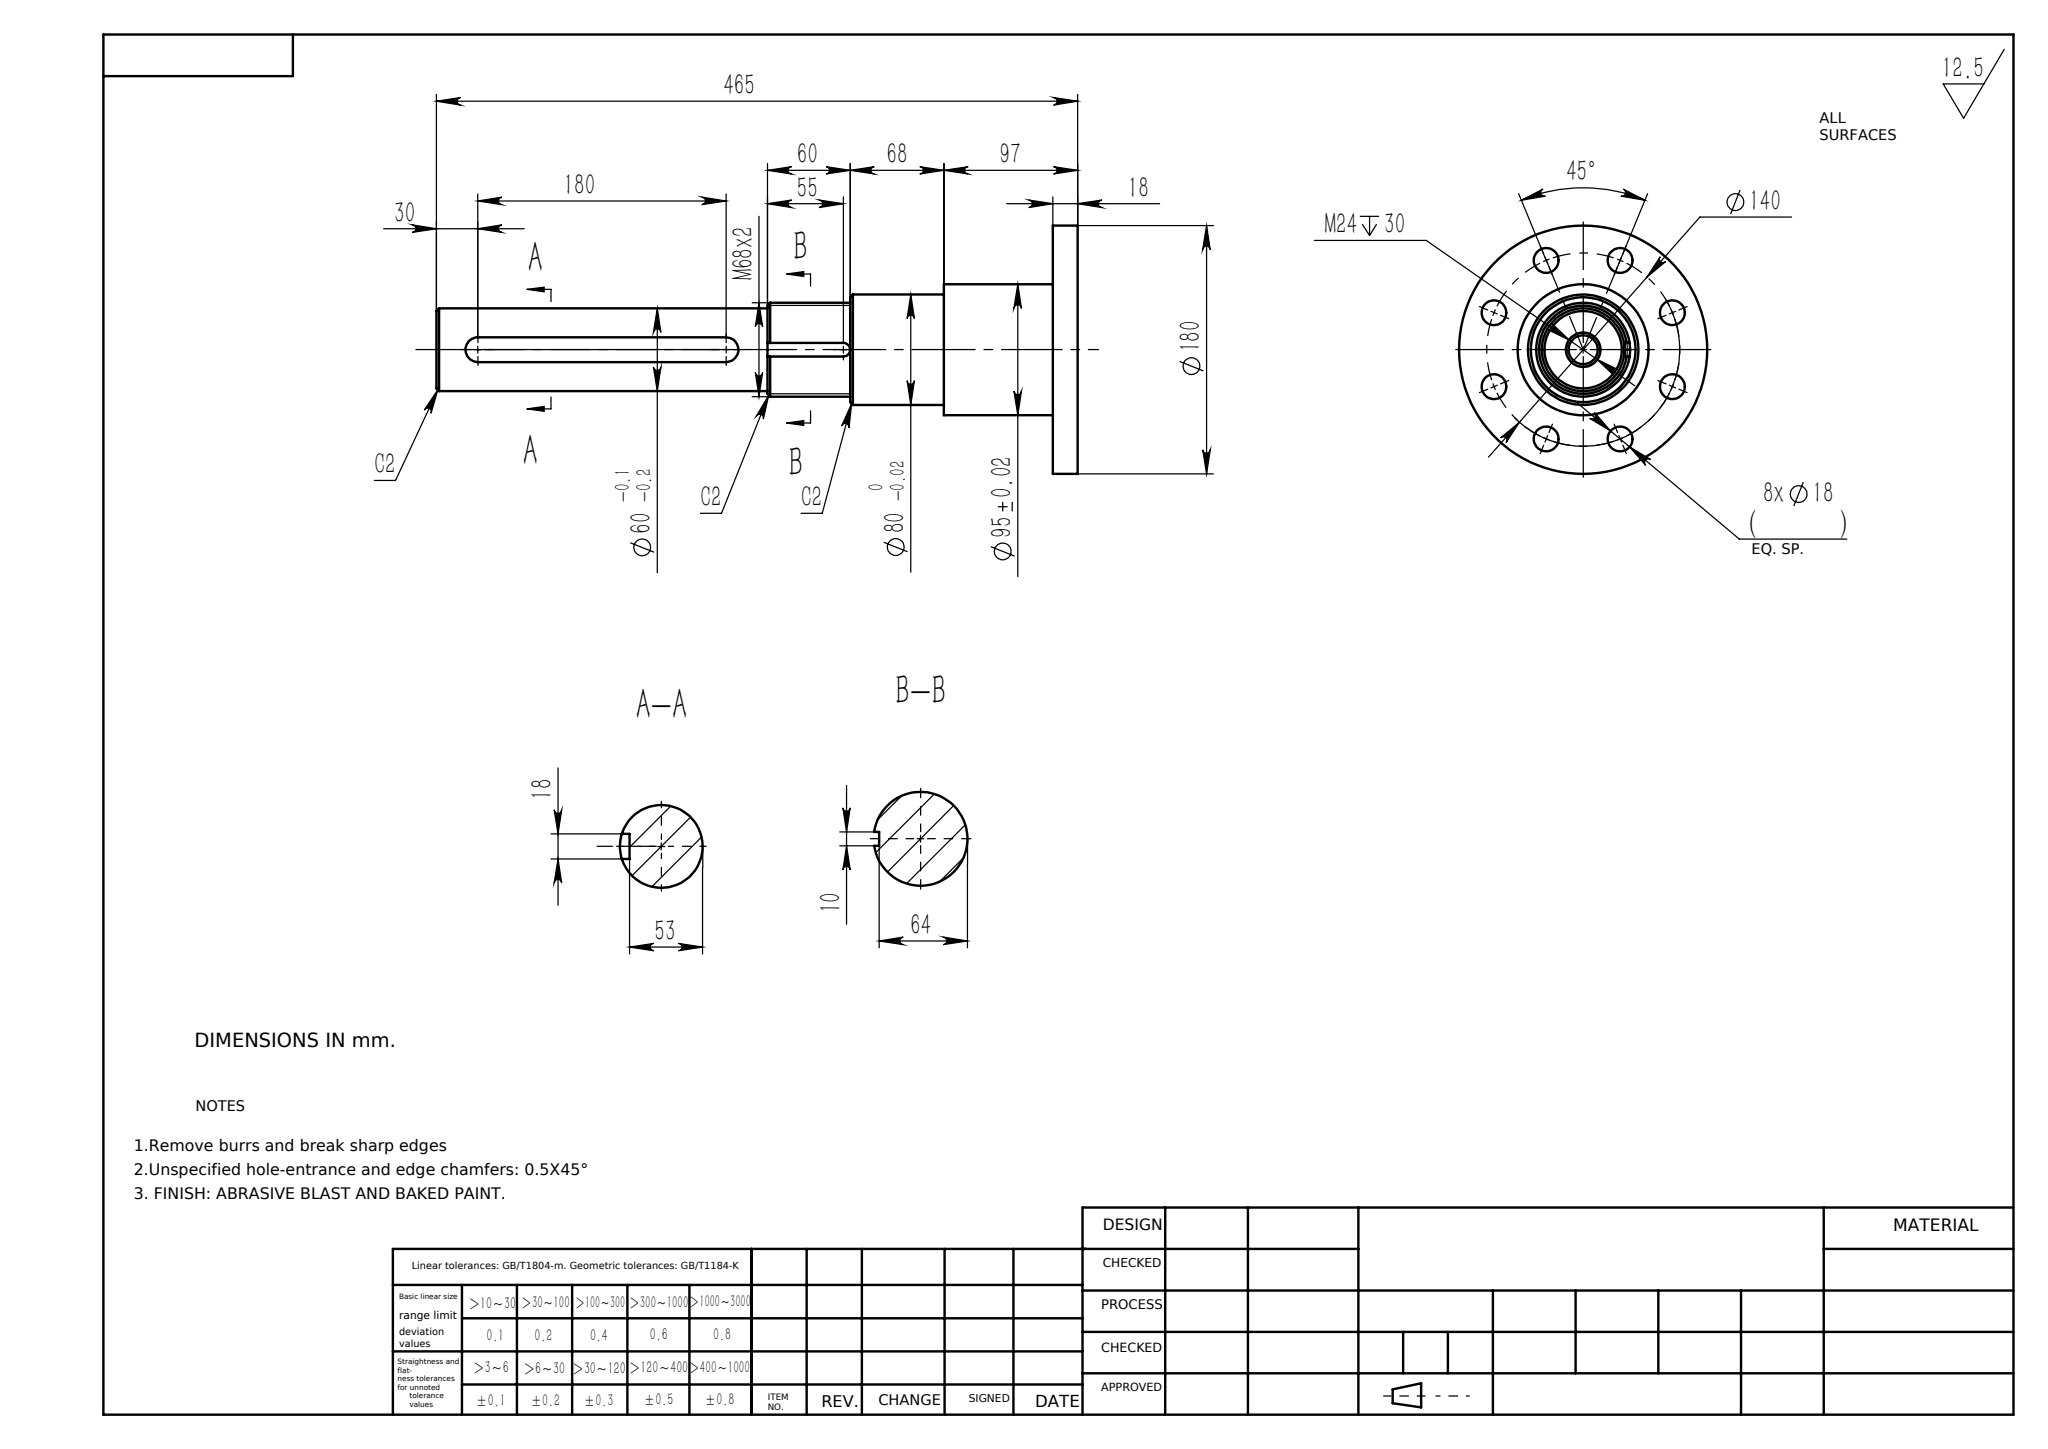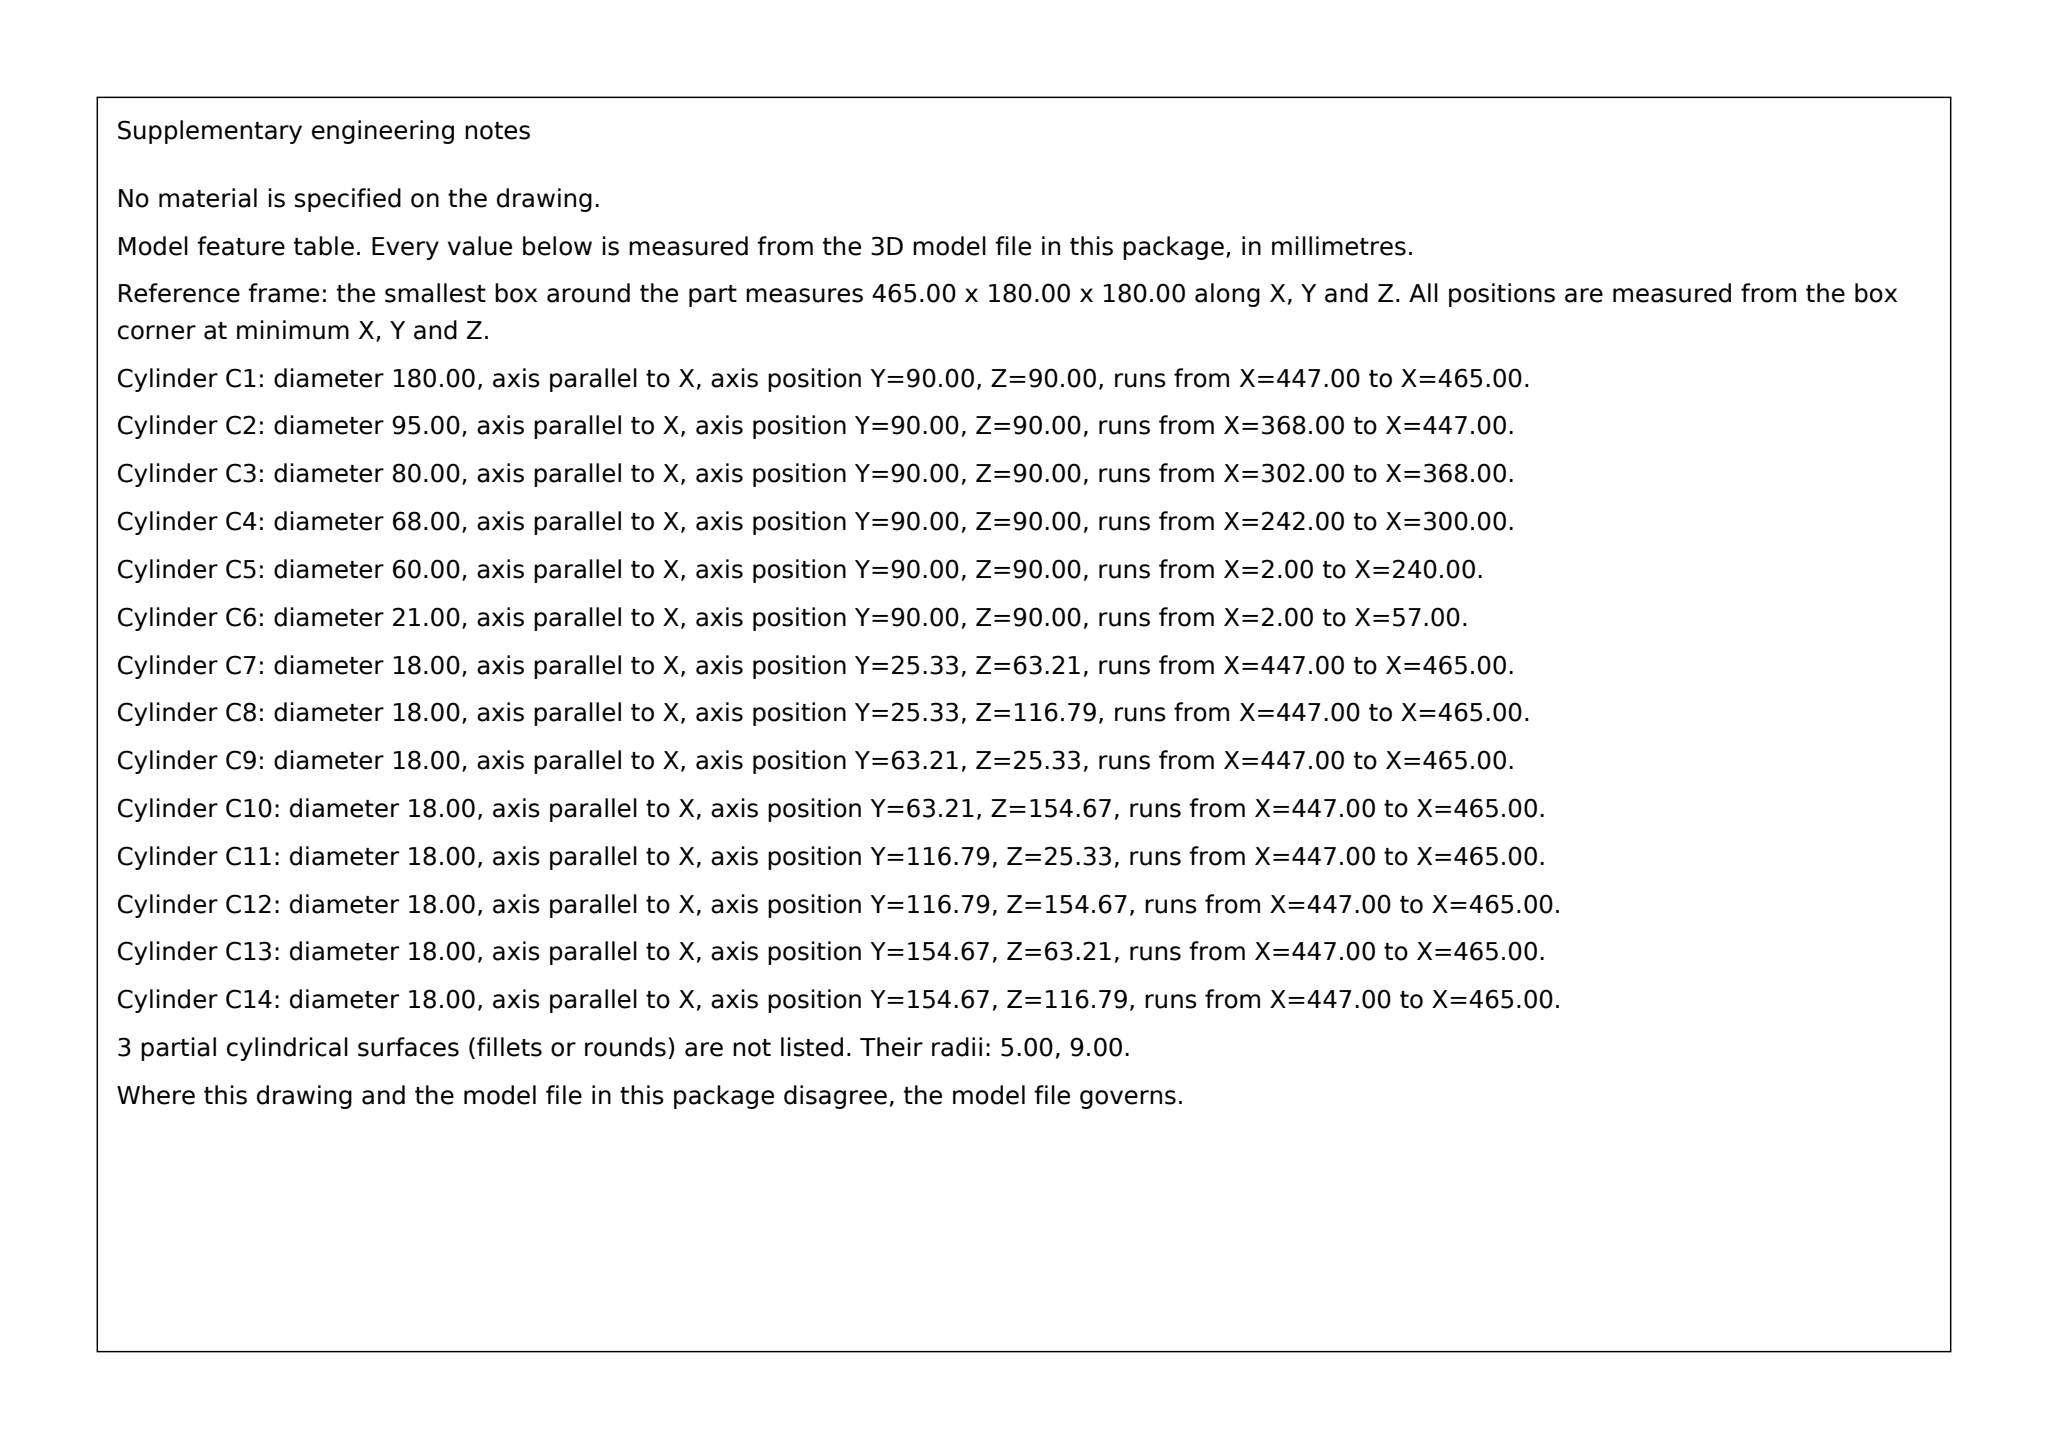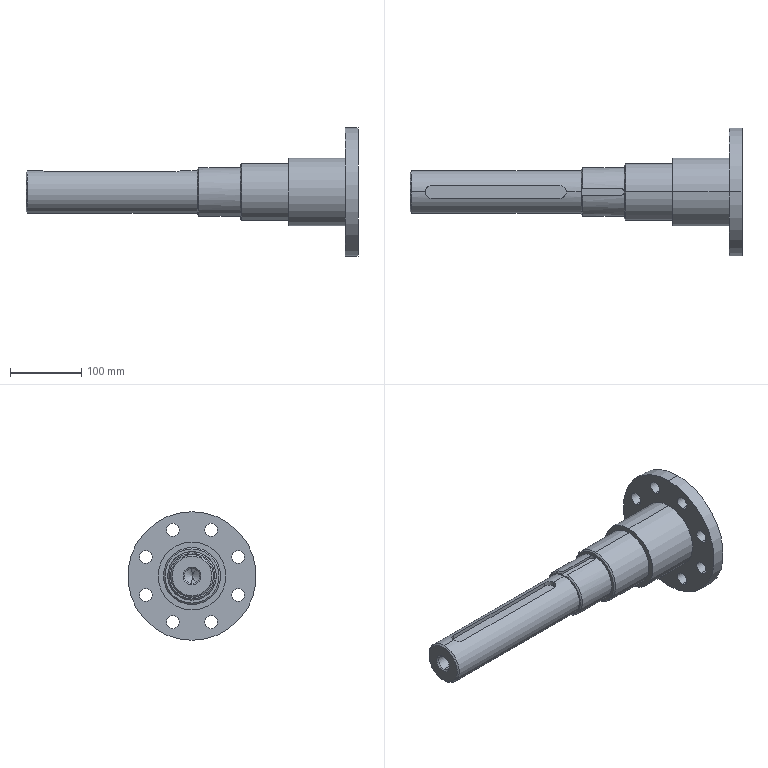Part | SolidWorks | mm | 1 solid | 55 faces | box 465 x 180 x 180 mm | volume 2172605 mm3 | cylinder 33 | plane 12 | cone 10 | commonest cylinder face diameters 18 x19 180 x2 21 x2 60 x2 68 x2 80 x2 95 x2 10 x2